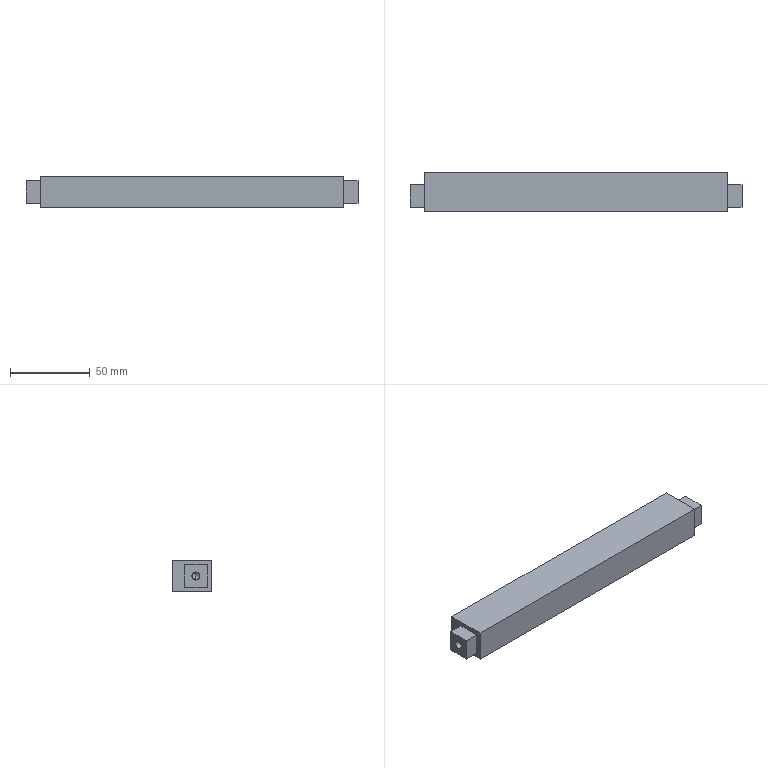Component | SolidWorks | Beam-1 | 1 solid | 38 faces | box 208 x 25 x 20 mm | volume 70503 mm3 | plane 22 | cone 8 | cylinder 8 | commonest cylinder face diameters 5 x4 10 x4
build123d program:
from build123d import *

# Parameters (mm, degrees)
SKETCH1_W           = 20
SKETCH1_H           = 25
BOSS_EXTRUDE1_DEPTH = 95
CUT_EXTRUDE4_DEPTH  = 20
SKETCH11_W          = 14
SKETCH11_H          = 14
BOSS_EXTRUDE3_DEPTH = 9


with BuildPart() as part:
    # Sketch1 → Boss-Extrude1 (new, symmetric)
    with BuildSketch(Plane(origin=(0, 0, 0), x_dir=(0, 0, -1), z_dir=(1, 0, 0))):
        with Locations((0, 20.347)):
            Rectangle(SKETCH1_W, SKETCH1_H)
    extrude(amount=BOSS_EXTRUDE1_DEPTH, both=True)

    # Sketch6 → Cut-Extrude4 (cut)
    with BuildSketch(Plane(origin=(0, 7.847, 0), x_dir=(-1, 0, 0), z_dir=(0, -1, 0))):
        with BuildLine():
            Line((75, -5), (15, -5))
            ThreePointArc((15, -5), (10, 0), (15, 5))
            Line((15, 5), (75, 5))
            ThreePointArc((75, 5), (80, 0), (75, -5))
        make_face()
        with BuildLine():
            Line((-75, -5), (-15, -5))
            ThreePointArc((-15, -5), (-10, 0), (-15, 5))
            Line((-15, 5), (-75, 5))
            ThreePointArc((-75, 5), (-80, 0), (-75, -5))
        make_face()
    extrude(amount=-CUT_EXTRUDE4_DEPTH, mode=Mode.SUBTRACT)

    # Sketch11 → Boss-Extrude3 (add)
    with BuildSketch(Plane(origin=(95, 0, 0), x_dir=(0, 0, -1), z_dir=(1, 0, 0))):
        with Locations((0, 22.847)):
            Rectangle(SKETCH11_W, SKETCH11_H)
    boss_extrude3 = extrude(amount=BOSS_EXTRUDE3_DEPTH)

    # Sketch12 → M5 Tapped Hole1 (revolve, cut)
    with BuildSketch(Plane(origin=(104, 22.847, 0), x_dir=(0, 0, -1), z_dir=(0, 1, 0))):
        Polygon((0, 0), (0, 23.502), (2.5, 22), (2.5, 0.025), (2.525, 0), align=None)
    m5_tapped_hole1 = revolve(axis=Axis((110.35, 22.847, 0), (-1, 0, 0)), mode=Mode.SUBTRACT)

    # Mirror1: Boss-Extrude3, M5 Tapped Hole1 across plane
    add(boss_extrude3.mirror(Plane(origin=(0, 0, 0), x_dir=(0, 0, 1), z_dir=(1, 0, 0))))
    add(m5_tapped_hole1.mirror(Plane(origin=(0, 0, 0), x_dir=(0, 0, 1), z_dir=(1, 0, 0))), mode=Mode.SUBTRACT)


solid = part.part

# Placed as in the assembly
solid = solid.moved(Location((-138.428, 50.643, 284.382), (180, 0, 0)))